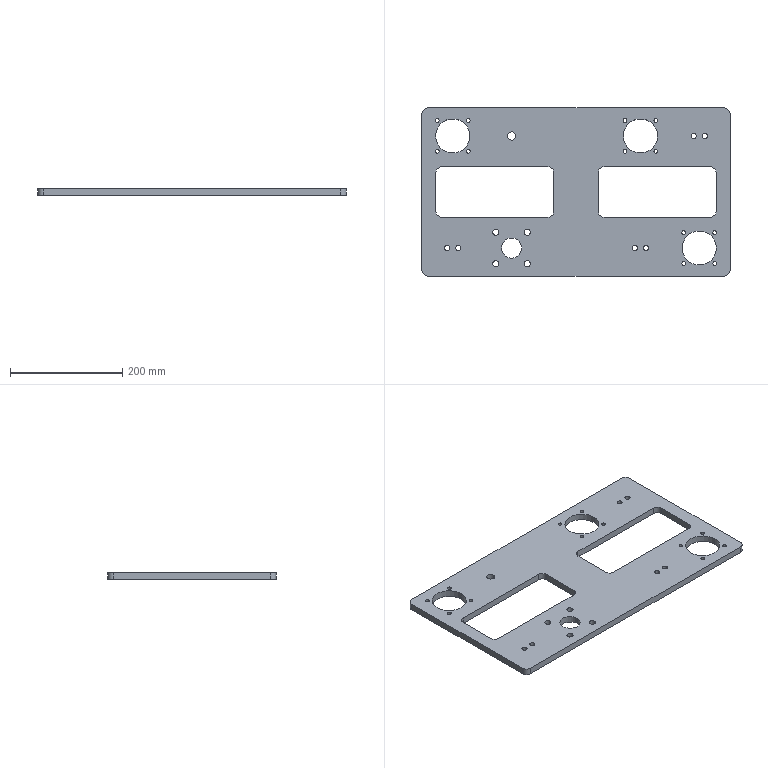Component | SolidWorks | CylinderPanel-1 | 1 solid | 80 faces | box 550 x 300 x 12 mm | volume 1393654 mm3 | cylinder 66 | plane 14 | commonest cylinder face diameters 6.8 x24 9 x12 20 x12 11 x8 61 x6 14.5 x2 36 x2 | material 6063
build123d program:
from build123d import *

# Parameters (mm, degrees)
SKETCH1_W                  = 550
SKETCH1_H                  = 300
BOSS_EXTRUDE1_DEPTH        = 12
FILLET1_R                  = 10
SKETCH8_W                  = 210
SKETCH8_H                  = 90
CUT_EXTRUDE4_DEPTH         = 314.479
FILLET2_R                  = 10
SKETCH12_R                 = 30.5
SKETCH12_R_2               = 18
SKETCH12_R_3               = 5.5
SKETCH12_R_4               = 4.5
CUT_EXTRUDE6_DEPTH         = 314.479
M8_TAPPED_HOLE1_D          = 6.8
M8_TAPPED_HOLE1_DEPTH      = 19.75
M8_TAPPED_HOLE1_TIP        = 2.043
M16X1_5_TAPPED_HOLE1_D     = 14.5
M16X1_5_TAPPED_HOLE1_DEPTH = 36.5
M16X1_5_TAPPED_HOLE1_TIP   = 4.356


with BuildPart() as part:
    # Sketch1 → Boss-Extrude1 (new body)
    with BuildSketch(Plane.XY):
        Rectangle(SKETCH1_W, SKETCH1_H)
    extrude(amount=BOSS_EXTRUDE1_DEPTH)

    # Fillet1
    fillet1_edges = [part.edges().sort_by_distance(p)[0] for p in [
        (275, -150, 6),
        (-275, -150, 6),
        (-275, 150, 6),
        (275, 150, 6),
    ]]
    fillet(fillet1_edges, radius=FILLET1_R)

    # Sketch8 → Cut-Extrude4 (cut, through all)
    with BuildSketch(Plane.XY.offset(12)):
        with Locations((145, 0)):
            Rectangle(SKETCH8_W, SKETCH8_H)
        with Locations((-145, 0)):
            Rectangle(SKETCH8_W, SKETCH8_H)
    extrude(amount=-CUT_EXTRUDE4_DEPTH, mode=Mode.SUBTRACT)

    # Fillet2
    fillet2_edges = [part.edges().sort_by_distance(p)[0] for p in [
        (250, 45, 6),
        (250, -45, 6),
        (40, -45, 6),
        (40, 45, 6),
        (-40, 45, 6),
        (-40, -45, 6),
        (-250, -45, 6),
        (-250, 45, 6),
    ]]
    fillet(fillet2_edges, radius=FILLET2_R)

    # Sketch12 → Cut-Extrude6 (cut, through all)
    with BuildSketch(Plane(origin=(0, 0, 0), x_dir=(-1, 0, 0), z_dir=(0, 0, -1))):
        with Locations((-220, -100)):
            Circle(SKETCH12_R)
        with Locations((220, 100)):
            Circle(SKETCH12_R)
        with Locations((-115, 100)):
            Circle(SKETCH12_R)
        with Locations((115, -100)):
            Circle(SKETCH12_R_2)
        with Locations((87, -72)):
            Circle(SKETCH12_R_3)
        with Locations((87, -128)):
            Circle(SKETCH12_R_3)
        with Locations((143, -128)):
            Circle(SKETCH12_R_3)
        with Locations((143, -72)):
            Circle(SKETCH12_R_3)
        with Locations((-230, 100)):
            Circle(SKETCH12_R_4)
        with Locations((-210, 100)):
            Circle(SKETCH12_R_4)
        with Locations((-125, -100)):
            Circle(SKETCH12_R_4)
        with Locations((-105, -100)):
            Circle(SKETCH12_R_4)
        with Locations((230, -100)):
            Circle(SKETCH12_R_4)
        with Locations((210, -100)):
            Circle(SKETCH12_R_4)
    extrude(amount=-CUT_EXTRUDE6_DEPTH, mode=Mode.SUBTRACT)

    # M8 Tapped Hole1
    with Locations(Plane(origin=(142.577, 127.577, 0), x_dir=(-1, 0, 0), z_dir=(0, 0, -1))):
        with Locations((0, 0), (55.154, 0), (55.154, -55.154), (0, -55.154), (335, 0), (390.154, 0), (390.154, -55.154), (335, -55.154), (-49.846, -200), (-105, -200), (-105, -255.154), (-49.846, -255.154)):
            Hole(M8_TAPPED_HOLE1_D / 2, depth=M8_TAPPED_HOLE1_DEPTH)
            with Locations((0, 0, -(M8_TAPPED_HOLE1_DEPTH + M8_TAPPED_HOLE1_TIP / 2))):  # 118° drill point
                Cone(0, M8_TAPPED_HOLE1_D / 2, M8_TAPPED_HOLE1_TIP, mode=Mode.SUBTRACT)

    # M16x1.5 Tapped Hole1
    with Locations(Plane(origin=(-115, 100, 0), x_dir=(-1, 0, 0), z_dir=(0, 0, -1))):
        with Locations((0, 0)):
            Hole(M16X1_5_TAPPED_HOLE1_D / 2, depth=M16X1_5_TAPPED_HOLE1_DEPTH)
            with Locations((0, 0, -(M16X1_5_TAPPED_HOLE1_DEPTH + M16X1_5_TAPPED_HOLE1_TIP / 2))):  # 118° drill point
                Cone(0, M16X1_5_TAPPED_HOLE1_D / 2, M16X1_5_TAPPED_HOLE1_TIP, mode=Mode.SUBTRACT)


solid = part.part

# Placed as in the assembly
solid = solid.moved(Location((1.785, 3.083, -796.191), (0, 0, 0)))